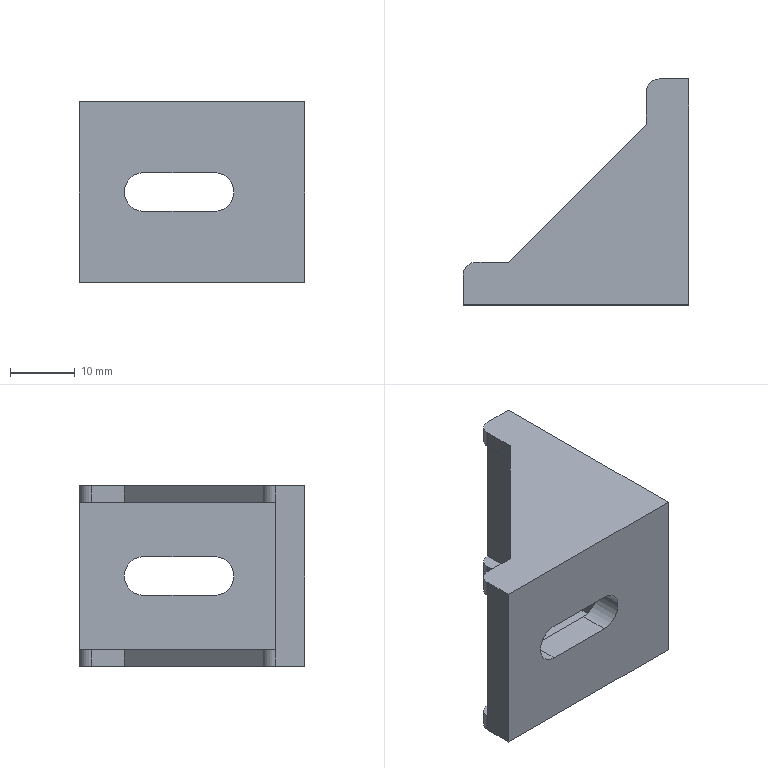Component | SolidWorks | Foot-1 | 1 solid | 28 faces | box 35 x 35 x 28 mm | volume 9349 mm3 | plane 20 | cylinder 8 | commonest cylinder face diameters 4 x4 6 x4
build123d program:
from build123d import *

# Parameters (mm, degrees)
BOSS_EXTRUDE1_DEPTH = 14
BOSS_EXTRUDE2_DEPTH = 2.6
FILLET1_R           = 2
CUT_EXTRUDE1_DEPTH  = 12.6
CUT_EXTRUDE2_DEPTH  = 12.6


with BuildPart() as part:
    # Sketch1 → Boss-Extrude1 (new, symmetric)
    with BuildSketch(Plane.XY):
        Polygon((0, 0), (35, 0), (35, 4.6), (4.6, 4.6), (4.6, 35), (0, 35), align=None)
    extrude(amount=BOSS_EXTRUDE1_DEPTH, both=True)

    # Sketch2 → Boss-Extrude2 (add)
    with BuildSketch(Plane.XY.offset(14)):
        Polygon((4.6, 35), (6.6, 35), (6.6, 28), (28, 6.6), (35, 6.6), (35, 4.6), (4.6, 4.6), align=None)
    boss_extrude2 = extrude(amount=-BOSS_EXTRUDE2_DEPTH)

    # Mirror1: Boss-Extrude2 across plane
    add(boss_extrude2.mirror(Plane.XY))

    # Fillet1
    fillet1_edges = [part.edges().sort_by_distance(p)[0] for p in [
        (35, 6.6, 12.7),
        (35, 6.6, -12.7),
        (6.6, 35, -12.7),
        (6.6, 35, 12.7),
    ]]
    fillet(fillet1_edges, radius=FILLET1_R)

    # Sketch3 → Cut-Extrude1 (cut)
    with BuildSketch(Plane(origin=(0, 4.6, 0), x_dir=(1, 0, 0), z_dir=(0, 1, 0))):
        with BuildLine():
            Line((14, 3), (25, 3))
            ThreePointArc((25, 3), (28, 0), (25, -3))
            Line((25, -3), (14, -3))
            ThreePointArc((14, -3), (11, 0), (14, 3))
        make_face()
    extrude(amount=-CUT_EXTRUDE1_DEPTH, mode=Mode.SUBTRACT)

    # Sketch4 → Cut-Extrude2 (cut)
    with BuildSketch(Plane(origin=(4.6, 0, 0), x_dir=(0, 0, -1), z_dir=(1, 0, 0))):
        with BuildLine():
            Line((3, 25), (3, 14))
            ThreePointArc((3, 14), (0, 11), (-3, 14))
            Line((-3, 14), (-3, 25))
            ThreePointArc((-3, 25), (0, 28), (3, 25))
        make_face()
    extrude(amount=-CUT_EXTRUDE2_DEPTH, mode=Mode.SUBTRACT)


solid = part.part

# Placed as in the assembly
solid = solid.moved(Location((80.237, -50.063, -152.804), (0, 0, 90)))